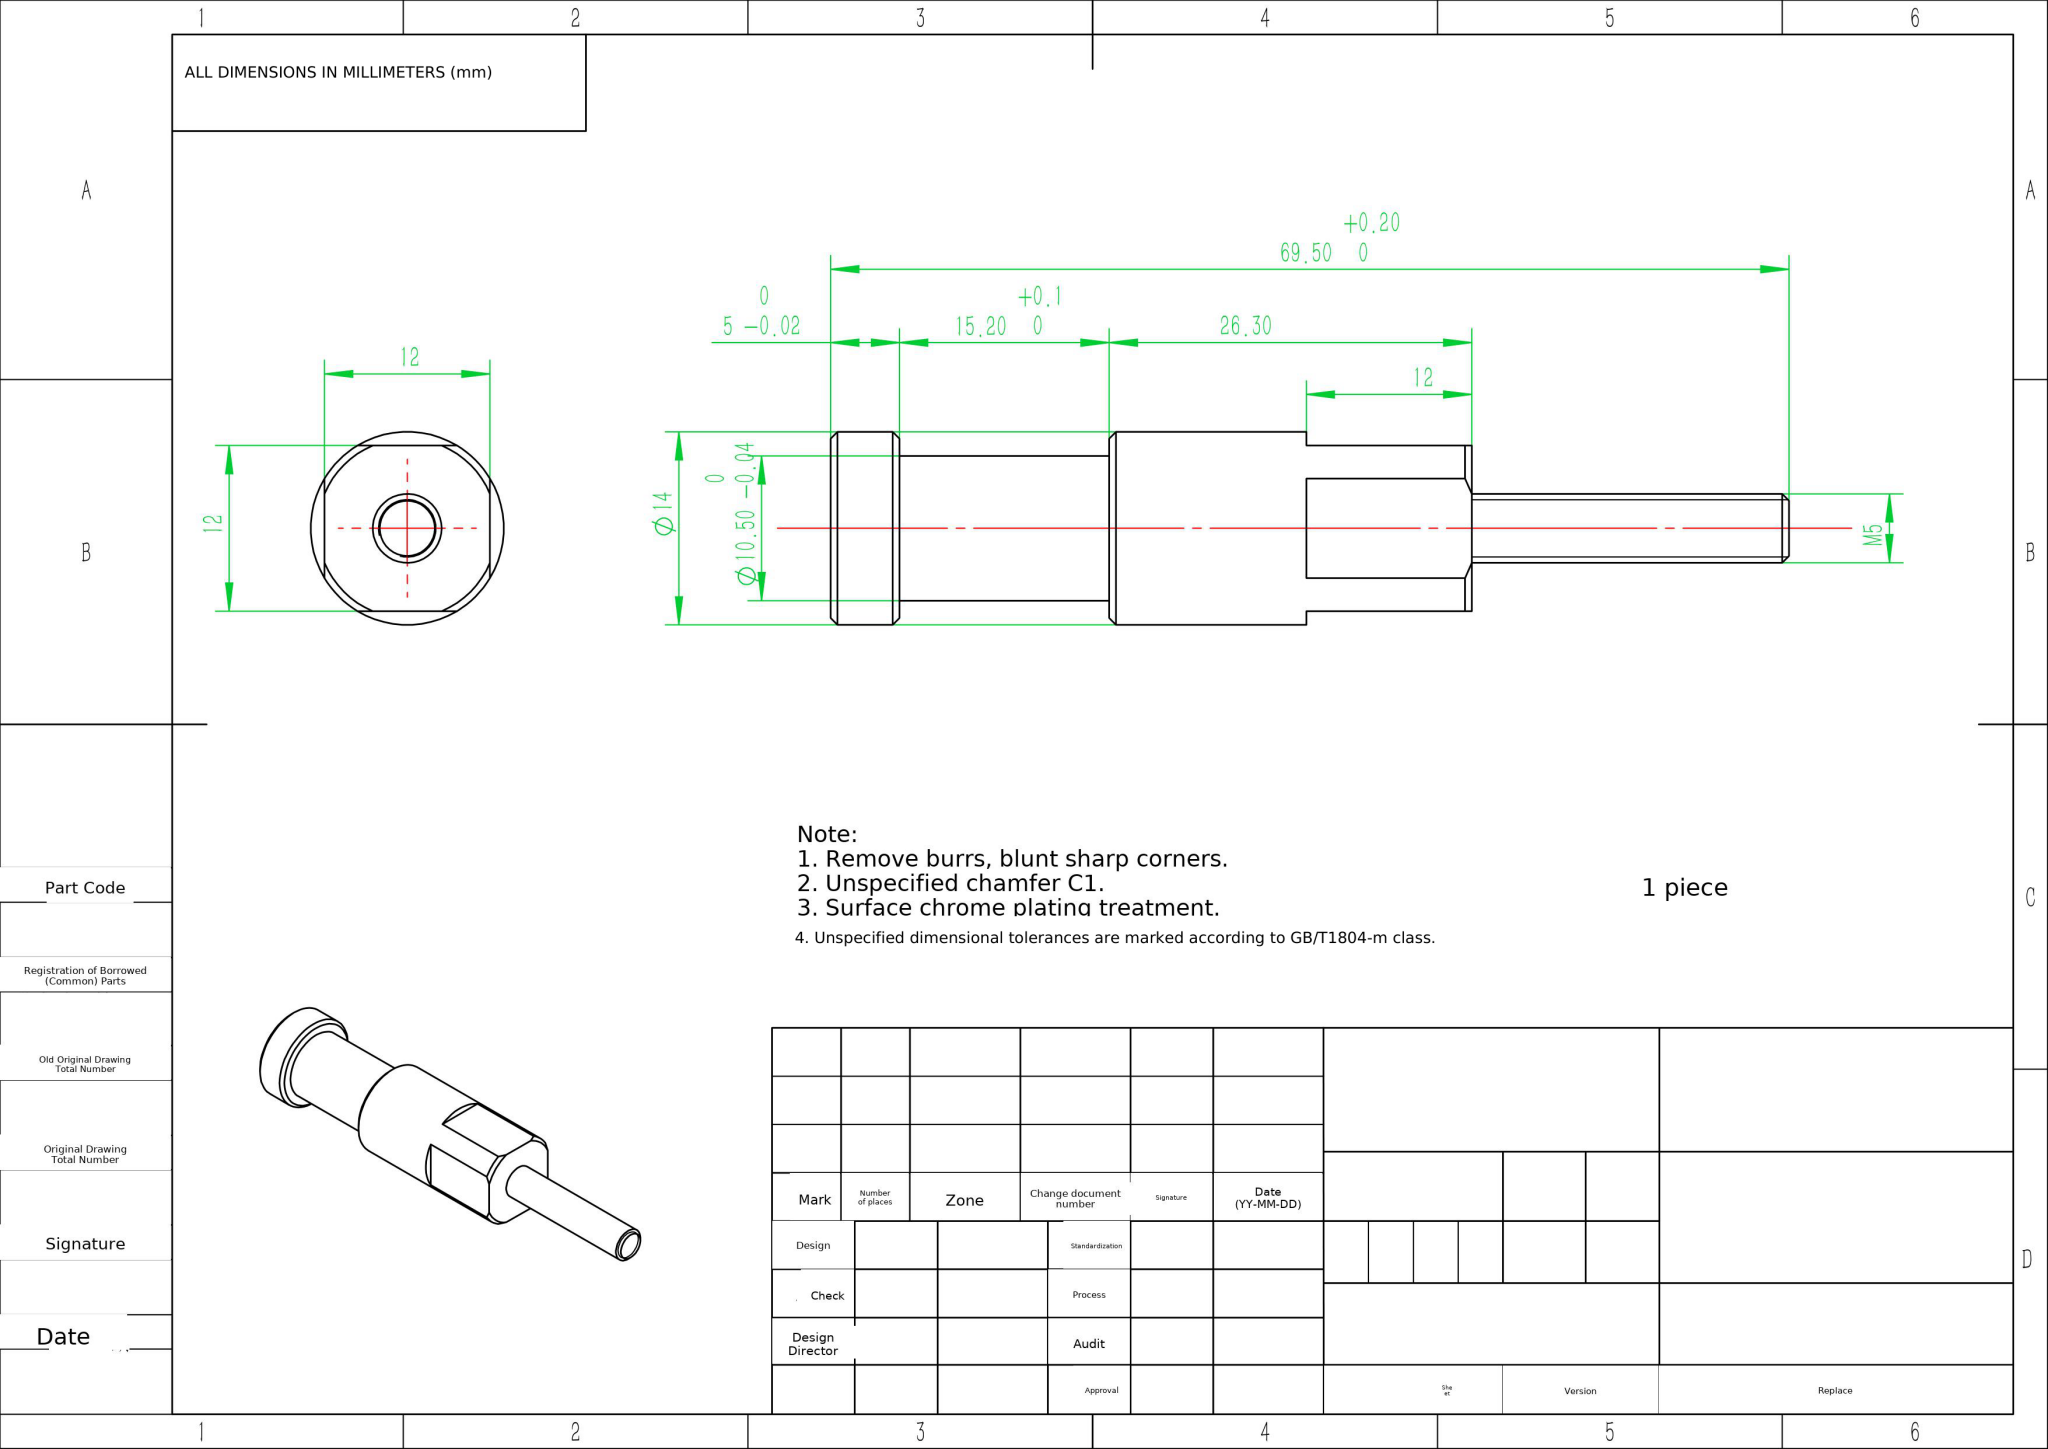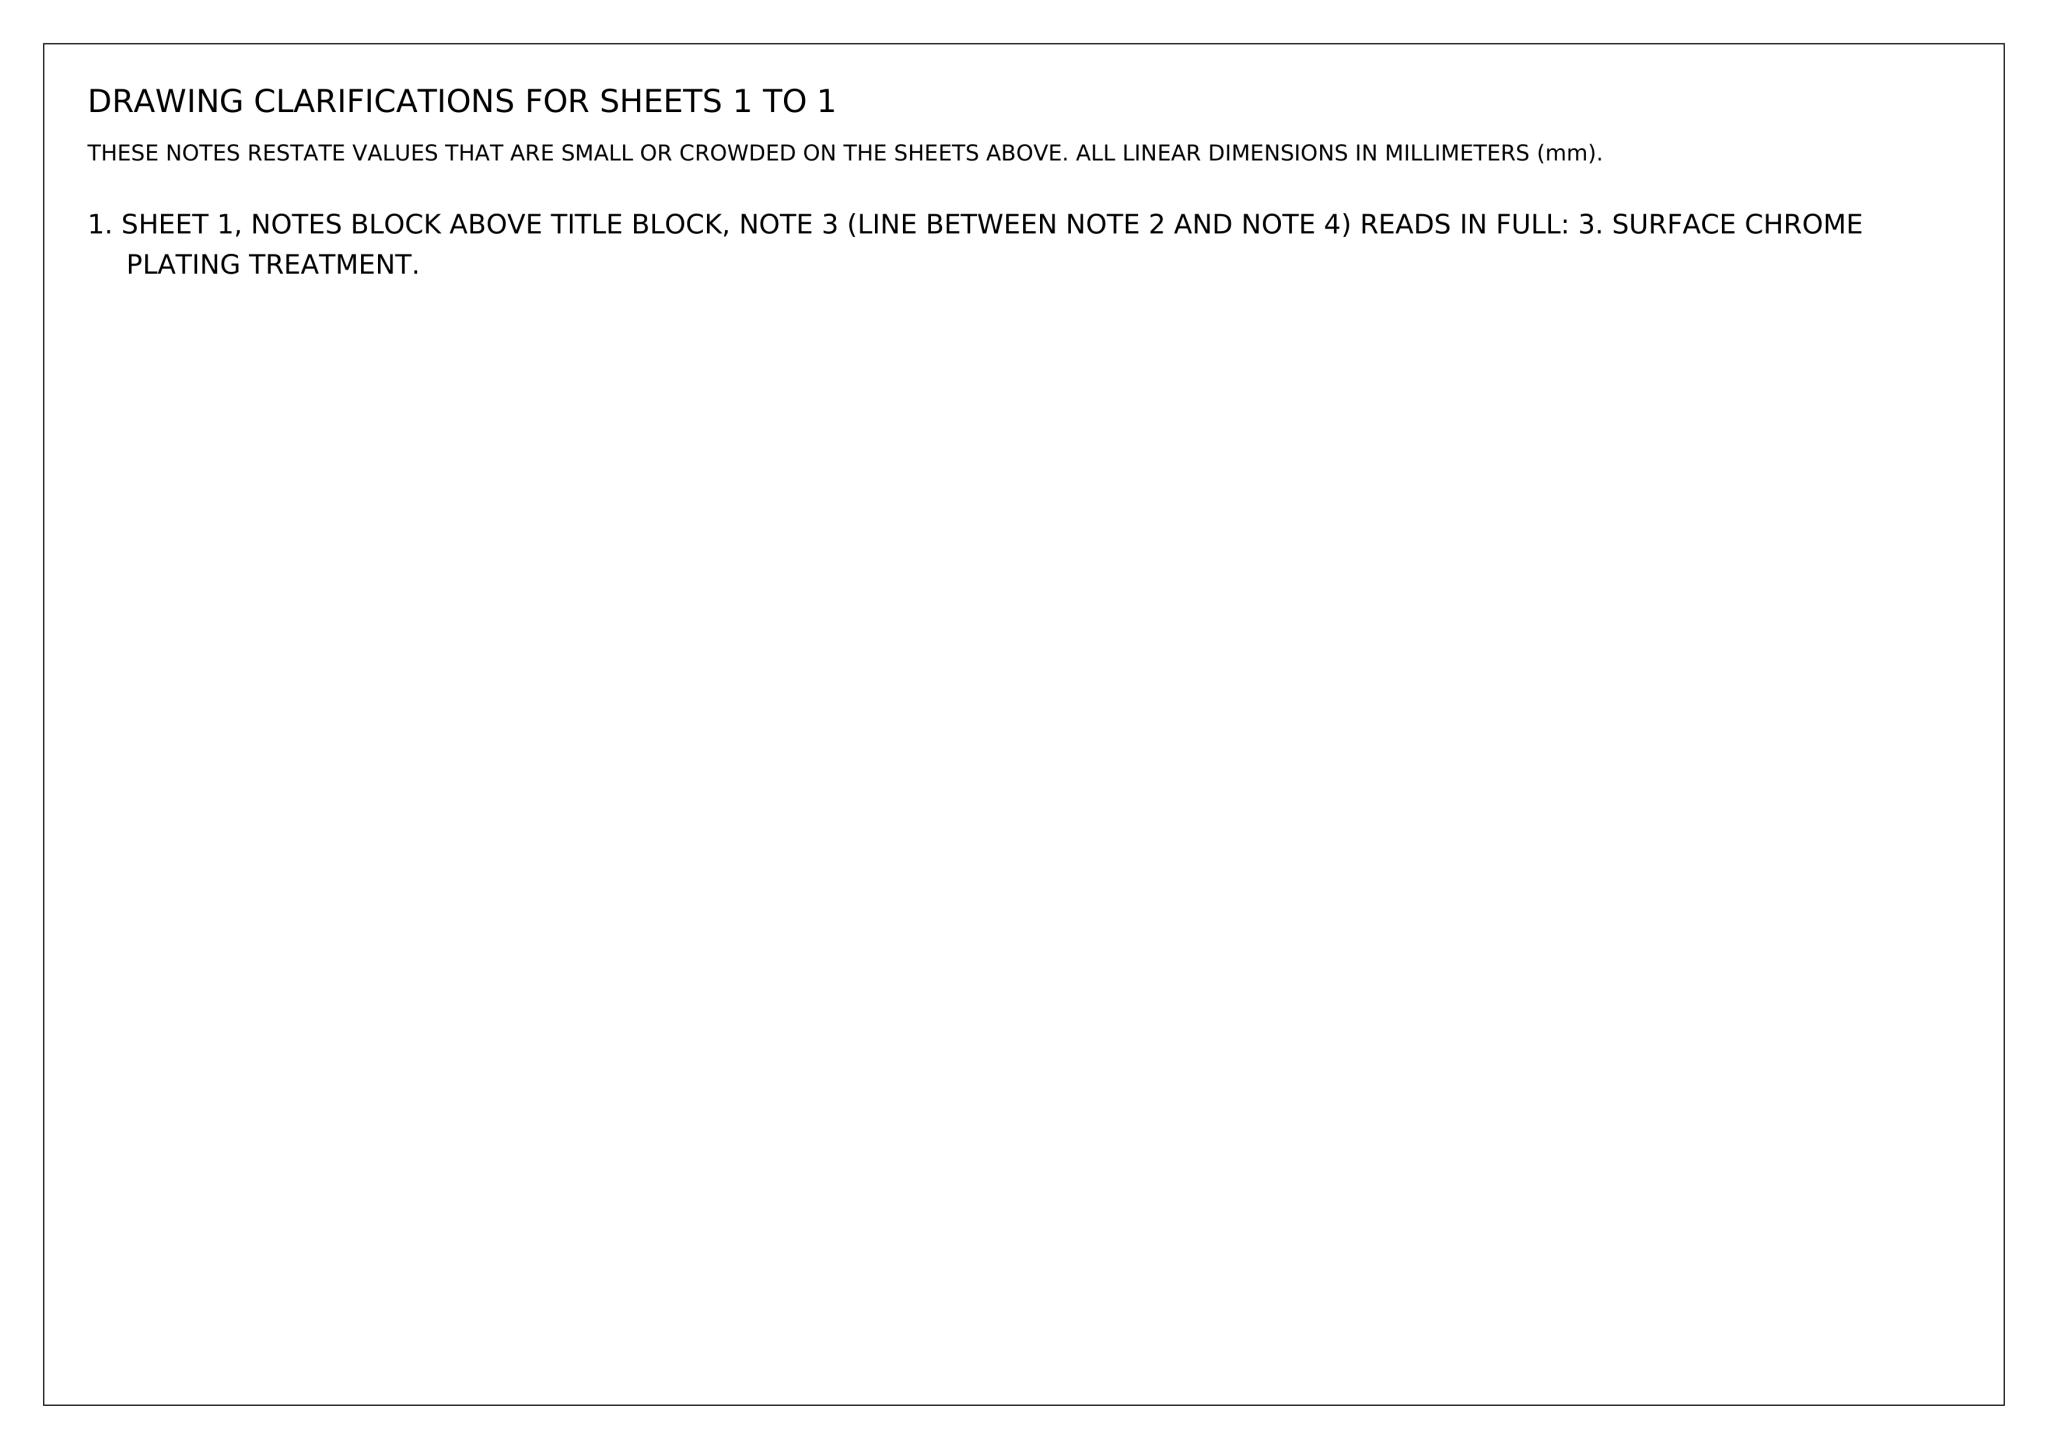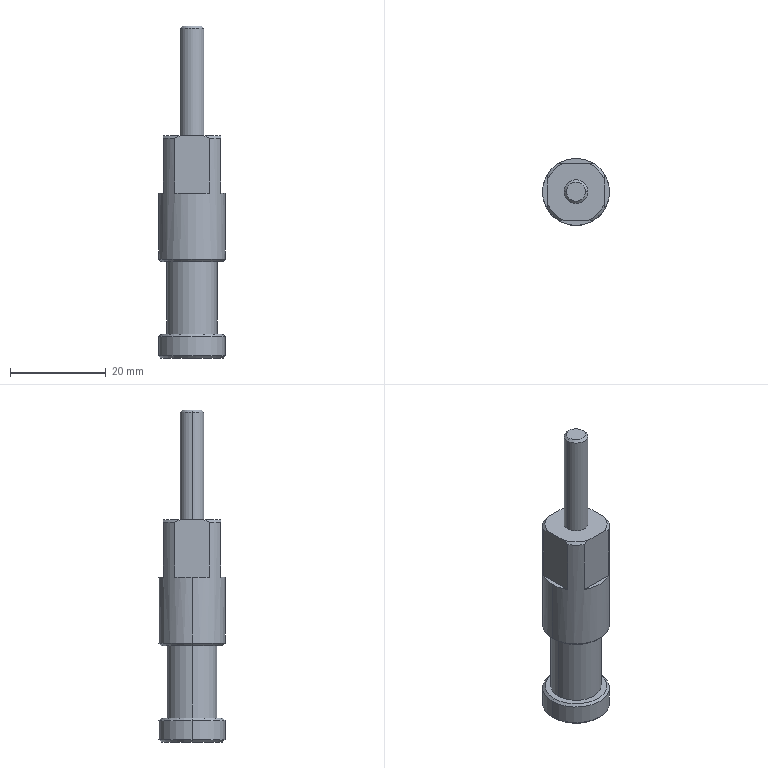Part | NX | mm | 1 solid | 33 faces | box 14 x 14 x 69.5 mm | volume 6332 mm3 | plane 13 | cone 12 | cylinder 8 | commonest cylinder face diameters 14 x4 5 x2 10.5 x2